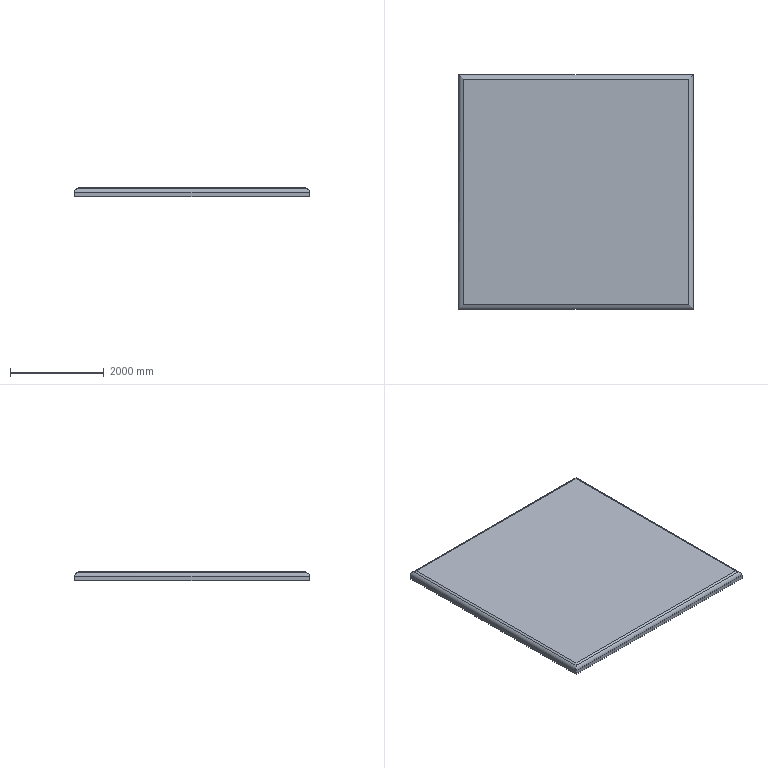Component | NX | 9_FLOOR | 1 solid | 14 faces | box 5000 x 5000 x 200 mm | volume 4937834897 mm3 | plane 10 | cylinder 4 | commonest cylinder face diameters 200 x4
STEP:
#1=CARTESIAN_POINT('',(0.,0.,0.));
#2=DIRECTION('',(0.,0.,1.));
#3=DIRECTION('',(1.,0.,0.));
#4=AXIS2_PLACEMENT_3D('',#1,#2,#3);
#5=CARTESIAN_POINT('',(3570.,2500.,-349.303));
#6=VERTEX_POINT('',#5);
#7=CARTESIAN_POINT('',(3570.,2500.,-437.5));
#8=VERTEX_POINT('',#7);
#9=CARTESIAN_POINT('',(3570.,2500.,-237.5));
#10=DIRECTION('',(0.,0.,-1.));
#11=VECTOR('',#10,1.);
#12=LINE('',#9,#11);
#13=CARTESIAN_POINT('',(3570.,-2500.,-237.5));
#14=DIRECTION('',(-1.,0.,0.));
#15=DIRECTION('',(-0.,-1.,0.));
#16=AXIS2_PLACEMENT_3D('',#13,#14,#15);
#17=PLANE('',#16);
#18=CARTESIAN_POINT('',(-5000.,0.));
#19=DIRECTION('',(0.,-1.));
#20=VECTOR('',#19,1.);
#21=LINE('',#18,#20);
#22=(GEOMETRIC_REPRESENTATION_CONTEXT(2)PARAMETRIC_REPRESENTATION_CONTEXT()REPRESENTATION_CONTEXT('',''));
#23=DEFINITIONAL_REPRESENTATION('',(#21),#22);
#24=PCURVE('',#17,#23);
#25=CARTESIAN_POINT('',(3570.,2500.,-237.5));
#26=DIRECTION('',(0.,-1.,0.));
#27=DIRECTION('',(0.,0.,1.));
#28=AXIS2_PLACEMENT_3D('',#25,#26,#27);
#29=PLANE('',#28);
#30=CARTESIAN_POINT('',(0.,0.));
#31=DIRECTION('',(-1.,0.));
#32=VECTOR('',#31,1.);
#33=LINE('',#30,#32);
#34=(GEOMETRIC_REPRESENTATION_CONTEXT(2)PARAMETRIC_REPRESENTATION_CONTEXT()REPRESENTATION_CONTEXT('',''));
#35=DEFINITIONAL_REPRESENTATION('',(#33),#34);
#36=PCURVE('',#29,#35);
#37=SURFACE_CURVE('',#12,(#24,#36),.PCURVE_S1.);
#38=EDGE_CURVE('',#6,#8,#37,.T.);
#39=ORIENTED_EDGE('',*,*,#38,.F.);
#40=CARTESIAN_POINT('',(3570.,-2500.,-349.303));
#41=VERTEX_POINT('',#40);
#42=CARTESIAN_POINT('',(3570.,-2500.,-349.303));
#43=DIRECTION('',(-0.,-1.,0.));
#44=VECTOR('',#43,1.);
#45=LINE('',#42,#44);
#46=CARTESIAN_POINT('',(0.,-111.803));
#47=DIRECTION('',(1.,0.));
#48=VECTOR('',#47,1.);
#49=LINE('',#46,#48);
#50=(GEOMETRIC_REPRESENTATION_CONTEXT(2)PARAMETRIC_REPRESENTATION_CONTEXT()REPRESENTATION_CONTEXT('',''));
#51=DEFINITIONAL_REPRESENTATION('',(#49),#50);
#52=PCURVE('',#17,#51);
#53=CARTESIAN_POINT('',(3470.,-2500.,-349.303));
#54=DIRECTION('',(0.,1.,0.));
#55=DIRECTION('',(-1.,0.,0.));
#56=AXIS2_PLACEMENT_3D('',#53,#54,#55);
#57=CYLINDRICAL_SURFACE('',#56,100.);
#58=CARTESIAN_POINT('',(3.142,0.));
#59=DIRECTION('',(0.,-1.));
#60=VECTOR('',#59,1.);
#61=LINE('',#58,#60);
#62=(GEOMETRIC_REPRESENTATION_CONTEXT(2)PARAMETRIC_REPRESENTATION_CONTEXT()REPRESENTATION_CONTEXT('',''));
#63=DEFINITIONAL_REPRESENTATION('',(#61),#62);
#64=PCURVE('',#57,#63);
#65=SURFACE_CURVE('',#45,(#52,#64),.PCURVE_S1.);
#66=EDGE_CURVE('',#6,#41,#65,.T.);
#67=ORIENTED_EDGE('',*,*,#66,.T.);
#68=CARTESIAN_POINT('',(3570.,-2500.,-437.5));
#69=VERTEX_POINT('',#68);
#70=CARTESIAN_POINT('',(3570.,-2500.,-237.5));
#71=DIRECTION('',(0.,0.,-1.));
#72=VECTOR('',#71,1.);
#73=LINE('',#70,#72);
#74=CARTESIAN_POINT('',(0.,0.));
#75=DIRECTION('',(0.,-1.));
#76=VECTOR('',#75,1.);
#77=LINE('',#74,#76);
#78=(GEOMETRIC_REPRESENTATION_CONTEXT(2)PARAMETRIC_REPRESENTATION_CONTEXT()REPRESENTATION_CONTEXT('',''));
#79=DEFINITIONAL_REPRESENTATION('',(#77),#78);
#80=PCURVE('',#17,#79);
#81=CARTESIAN_POINT('',(-1430.,-2500.,-237.5));
#82=DIRECTION('',(0.,1.,0.));
#83=DIRECTION('',(0.,0.,-1.));
#84=AXIS2_PLACEMENT_3D('',#81,#82,#83);
#85=PLANE('',#84);
#86=CARTESIAN_POINT('',(0.,-5000.));
#87=DIRECTION('',(1.,0.));
#88=VECTOR('',#87,1.);
#89=LINE('',#86,#88);
#90=(GEOMETRIC_REPRESENTATION_CONTEXT(2)PARAMETRIC_REPRESENTATION_CONTEXT()REPRESENTATION_CONTEXT('',''));
#91=DEFINITIONAL_REPRESENTATION('',(#89),#90);
#92=PCURVE('',#85,#91);
#93=SURFACE_CURVE('',#73,(#80,#92),.PCURVE_S1.);
#94=EDGE_CURVE('',#41,#69,#93,.T.);
#95=ORIENTED_EDGE('',*,*,#94,.T.);
#96=CARTESIAN_POINT('',(3570.,-2500.,-437.5));
#97=DIRECTION('',(0.,1.,0.));
#98=VECTOR('',#97,1.);
#99=LINE('',#96,#98);
#100=CARTESIAN_POINT('',(0.,-200.));
#101=DIRECTION('',(-1.,0.));
#102=VECTOR('',#101,1.);
#103=LINE('',#100,#102);
#104=(GEOMETRIC_REPRESENTATION_CONTEXT(2)PARAMETRIC_REPRESENTATION_CONTEXT()REPRESENTATION_CONTEXT('',''));
#105=DEFINITIONAL_REPRESENTATION('',(#103),#104);
#106=PCURVE('',#17,#105);
#107=CARTESIAN_POINT('',(1070.,-0.,-437.5));
#108=DIRECTION('',(0.,0.,1.));
#109=DIRECTION('',(-1.,0.,0.));
#110=AXIS2_PLACEMENT_3D('',#107,#108,#109);
#111=PLANE('',#110);
#112=CARTESIAN_POINT('',(-2500.,2500.));
#113=DIRECTION('',(-0.,-1.));
#114=VECTOR('',#113,1.);
#115=LINE('',#112,#114);
#116=(GEOMETRIC_REPRESENTATION_CONTEXT(2)PARAMETRIC_REPRESENTATION_CONTEXT()REPRESENTATION_CONTEXT('',''));
#117=DEFINITIONAL_REPRESENTATION('',(#115),#116);
#118=PCURVE('',#111,#117);
#119=SURFACE_CURVE('',#99,(#106,#118),.PCURVE_S1.);
#120=EDGE_CURVE('',#69,#8,#119,.T.);
#121=ORIENTED_EDGE('',*,*,#120,.T.);
#122=EDGE_LOOP('',(#39,#67,#95,#121));
#123=FACE_BOUND('',#122,.T.);
#124=ADVANCED_FACE('',(#123),#17,.F.);
#125=CARTESIAN_POINT('',(-1430.,2500.,-349.303));
#126=VERTEX_POINT('',#125);
#127=CARTESIAN_POINT('',(-1430.,2500.,-437.5));
#128=VERTEX_POINT('',#127);
#129=CARTESIAN_POINT('',(-1430.,2500.,-237.5));
#130=DIRECTION('',(0.,0.,-1.));
#131=VECTOR('',#130,1.);
#132=LINE('',#129,#131);
#133=CARTESIAN_POINT('',(0.,5000.));
#134=DIRECTION('',(-1.,0.));
#135=VECTOR('',#134,1.);
#136=LINE('',#133,#135);
#137=(GEOMETRIC_REPRESENTATION_CONTEXT(2)PARAMETRIC_REPRESENTATION_CONTEXT()REPRESENTATION_CONTEXT('',''));
#138=DEFINITIONAL_REPRESENTATION('',(#136),#137);
#139=PCURVE('',#29,#138);
#140=CARTESIAN_POINT('',(-1430.,2500.,-237.5));
#141=DIRECTION('',(1.,-0.,0.));
#142=DIRECTION('',(0.,1.,0.));
#143=AXIS2_PLACEMENT_3D('',#140,#141,#142);
#144=PLANE('',#143);
#145=CARTESIAN_POINT('',(0.,0.));
#146=DIRECTION('',(0.,-1.));
#147=VECTOR('',#146,1.);
#148=LINE('',#145,#147);
#149=(GEOMETRIC_REPRESENTATION_CONTEXT(2)PARAMETRIC_REPRESENTATION_CONTEXT()REPRESENTATION_CONTEXT('',''));
#150=DEFINITIONAL_REPRESENTATION('',(#148),#149);
#151=PCURVE('',#144,#150);
#152=SURFACE_CURVE('',#132,(#139,#151),.PCURVE_S1.);
#153=EDGE_CURVE('',#126,#128,#152,.T.);
#154=ORIENTED_EDGE('',*,*,#153,.F.);
#155=CARTESIAN_POINT('',(3570.,2500.,-349.303));
#156=DIRECTION('',(1.,0.,0.));
#157=VECTOR('',#156,1.);
#158=LINE('',#155,#157);
#159=CARTESIAN_POINT('',(-111.803,0.));
#160=DIRECTION('',(0.,-1.));
#161=VECTOR('',#160,1.);
#162=LINE('',#159,#161);
#163=(GEOMETRIC_REPRESENTATION_CONTEXT(2)PARAMETRIC_REPRESENTATION_CONTEXT()REPRESENTATION_CONTEXT('',''));
#164=DEFINITIONAL_REPRESENTATION('',(#162),#163);
#165=PCURVE('',#29,#164);
#166=CARTESIAN_POINT('',(3570.,2400.,-349.303));
#167=DIRECTION('',(-1.,0.,0.));
#168=DIRECTION('',(0.,0.,-1.));
#169=AXIS2_PLACEMENT_3D('',#166,#167,#168);
#170=CYLINDRICAL_SURFACE('',#169,100.);
#171=CARTESIAN_POINT('',(4.712,0.));
#172=DIRECTION('',(0.,-1.));
#173=VECTOR('',#172,1.);
#174=LINE('',#171,#173);
#175=(GEOMETRIC_REPRESENTATION_CONTEXT(2)PARAMETRIC_REPRESENTATION_CONTEXT()REPRESENTATION_CONTEXT('',''));
#176=DEFINITIONAL_REPRESENTATION('',(#174),#175);
#177=PCURVE('',#170,#176);
#178=SURFACE_CURVE('',#158,(#165,#177),.PCURVE_S1.);
#179=EDGE_CURVE('',#126,#6,#178,.T.);
#180=ORIENTED_EDGE('',*,*,#179,.T.);
#181=ORIENTED_EDGE('',*,*,#38,.T.);
#182=CARTESIAN_POINT('',(3570.,2500.,-437.5));
#183=DIRECTION('',(-1.,0.,0.));
#184=VECTOR('',#183,1.);
#185=LINE('',#182,#184);
#186=CARTESIAN_POINT('',(-200.,0.));
#187=DIRECTION('',(0.,1.));
#188=VECTOR('',#187,1.);
#189=LINE('',#186,#188);
#190=(GEOMETRIC_REPRESENTATION_CONTEXT(2)PARAMETRIC_REPRESENTATION_CONTEXT()REPRESENTATION_CONTEXT('',''));
#191=DEFINITIONAL_REPRESENTATION('',(#189),#190);
#192=PCURVE('',#29,#191);
#193=CARTESIAN_POINT('',(-2500.,-2500.));
#194=DIRECTION('',(1.,0.));
#195=VECTOR('',#194,1.);
#196=LINE('',#193,#195);
#197=(GEOMETRIC_REPRESENTATION_CONTEXT(2)PARAMETRIC_REPRESENTATION_CONTEXT()REPRESENTATION_CONTEXT('',''));
#198=DEFINITIONAL_REPRESENTATION('',(#196),#197);
#199=PCURVE('',#111,#198);
#200=SURFACE_CURVE('',#185,(#192,#199),.PCURVE_S1.);
#201=EDGE_CURVE('',#8,#128,#200,.T.);
#202=ORIENTED_EDGE('',*,*,#201,.T.);
#203=EDGE_LOOP('',(#154,#180,#181,#202));
#204=FACE_BOUND('',#203,.T.);
#205=ADVANCED_FACE('',(#204),#29,.F.);
#206=CARTESIAN_POINT('',(-1430.,-2500.,-349.303));
#207=VERTEX_POINT('',#206);
#208=CARTESIAN_POINT('',(-1430.,-2500.,-437.5));
#209=VERTEX_POINT('',#208);
#210=CARTESIAN_POINT('',(-1430.,-2500.,-237.5));
#211=DIRECTION('',(0.,0.,-1.));
#212=VECTOR('',#211,1.);
#213=LINE('',#210,#212);
#214=CARTESIAN_POINT('',(-5000.,0.));
#215=DIRECTION('',(0.,-1.));
#216=VECTOR('',#215,1.);
#217=LINE('',#214,#216);
#218=(GEOMETRIC_REPRESENTATION_CONTEXT(2)PARAMETRIC_REPRESENTATION_CONTEXT()REPRESENTATION_CONTEXT('',''));
#219=DEFINITIONAL_REPRESENTATION('',(#217),#218);
#220=PCURVE('',#144,#219);
#221=CARTESIAN_POINT('',(0.,0.));
#222=DIRECTION('',(1.,0.));
#223=VECTOR('',#222,1.);
#224=LINE('',#221,#223);
#225=(GEOMETRIC_REPRESENTATION_CONTEXT(2)PARAMETRIC_REPRESENTATION_CONTEXT()REPRESENTATION_CONTEXT('',''));
#226=DEFINITIONAL_REPRESENTATION('',(#224),#225);
#227=PCURVE('',#85,#226);
#228=SURFACE_CURVE('',#213,(#220,#227),.PCURVE_S1.);
#229=EDGE_CURVE('',#207,#209,#228,.T.);
#230=ORIENTED_EDGE('',*,*,#229,.F.);
#231=CARTESIAN_POINT('',(-1430.,2500.,-349.303));
#232=DIRECTION('',(0.,1.,0.));
#233=VECTOR('',#232,1.);
#234=LINE('',#231,#233);
#235=CARTESIAN_POINT('',(0.,-111.803));
#236=DIRECTION('',(1.,0.));
#237=VECTOR('',#236,1.);
#238=LINE('',#235,#237);
#239=(GEOMETRIC_REPRESENTATION_CONTEXT(2)PARAMETRIC_REPRESENTATION_CONTEXT()REPRESENTATION_CONTEXT('',''));
#240=DEFINITIONAL_REPRESENTATION('',(#238),#239);
#241=PCURVE('',#144,#240);
#242=CARTESIAN_POINT('',(-1330.,2500.,-349.303));
#243=DIRECTION('',(-0.,-1.,0.));
#244=DIRECTION('',(1.,-0.,0.));
#245=AXIS2_PLACEMENT_3D('',#242,#243,#244);
#246=CYLINDRICAL_SURFACE('',#245,100.);
#247=CARTESIAN_POINT('',(3.142,0.));
#248=DIRECTION('',(0.,-1.));
#249=VECTOR('',#248,1.);
#250=LINE('',#247,#249);
#251=(GEOMETRIC_REPRESENTATION_CONTEXT(2)PARAMETRIC_REPRESENTATION_CONTEXT()REPRESENTATION_CONTEXT('',''));
#252=DEFINITIONAL_REPRESENTATION('',(#250),#251);
#253=PCURVE('',#246,#252);
#254=SURFACE_CURVE('',#234,(#241,#253),.PCURVE_S1.);
#255=EDGE_CURVE('',#207,#126,#254,.T.);
#256=ORIENTED_EDGE('',*,*,#255,.T.);
#257=ORIENTED_EDGE('',*,*,#153,.T.);
#258=CARTESIAN_POINT('',(-1430.,2500.,-437.5));
#259=DIRECTION('',(-0.,-1.,0.));
#260=VECTOR('',#259,1.);
#261=LINE('',#258,#260);
#262=CARTESIAN_POINT('',(0.,-200.));
#263=DIRECTION('',(-1.,0.));
#264=VECTOR('',#263,1.);
#265=LINE('',#262,#264);
#266=(GEOMETRIC_REPRESENTATION_CONTEXT(2)PARAMETRIC_REPRESENTATION_CONTEXT()REPRESENTATION_CONTEXT('',''));
#267=DEFINITIONAL_REPRESENTATION('',(#265),#266);
#268=PCURVE('',#144,#267);
#269=CARTESIAN_POINT('',(2500.,-2500.));
#270=DIRECTION('',(0.,1.));
#271=VECTOR('',#270,1.);
#272=LINE('',#269,#271);
#273=(GEOMETRIC_REPRESENTATION_CONTEXT(2)PARAMETRIC_REPRESENTATION_CONTEXT()REPRESENTATION_CONTEXT('',''));
#274=DEFINITIONAL_REPRESENTATION('',(#272),#273);
#275=PCURVE('',#111,#274);
#276=SURFACE_CURVE('',#261,(#268,#275),.PCURVE_S1.);
#277=EDGE_CURVE('',#128,#209,#276,.T.);
#278=ORIENTED_EDGE('',*,*,#277,.T.);
#279=EDGE_LOOP('',(#230,#256,#257,#278));
#280=FACE_BOUND('',#279,.T.);
#281=ADVANCED_FACE('',(#280),#144,.F.);
#282=ORIENTED_EDGE('',*,*,#94,.F.);
#283=CARTESIAN_POINT('',(-1430.,-2500.,-349.303));
#284=DIRECTION('',(-1.,0.,0.));
#285=VECTOR('',#284,1.);
#286=LINE('',#283,#285);
#287=CARTESIAN_POINT('',(111.803,0.));
#288=DIRECTION('',(0.,1.));
#289=VECTOR('',#288,1.);
#290=LINE('',#287,#289);
#291=(GEOMETRIC_REPRESENTATION_CONTEXT(2)PARAMETRIC_REPRESENTATION_CONTEXT()REPRESENTATION_CONTEXT('',''));
#292=DEFINITIONAL_REPRESENTATION('',(#290),#291);
#293=PCURVE('',#85,#292);
#294=CARTESIAN_POINT('',(-1430.,-2400.,-349.303));
#295=DIRECTION('',(1.,0.,0.));
#296=DIRECTION('',(0.,0.,1.));
#297=AXIS2_PLACEMENT_3D('',#294,#295,#296);
#298=CYLINDRICAL_SURFACE('',#297,100.);
#299=CARTESIAN_POINT('',(1.571,0.));
#300=DIRECTION('',(0.,-1.));
#301=VECTOR('',#300,1.);
#302=LINE('',#299,#301);
#303=(GEOMETRIC_REPRESENTATION_CONTEXT(2)PARAMETRIC_REPRESENTATION_CONTEXT()REPRESENTATION_CONTEXT('',''));
#304=DEFINITIONAL_REPRESENTATION('',(#302),#303);
#305=PCURVE('',#298,#304);
#306=SURFACE_CURVE('',#286,(#293,#305),.PCURVE_S1.);
#307=EDGE_CURVE('',#41,#207,#306,.T.);
#308=ORIENTED_EDGE('',*,*,#307,.T.);
#309=ORIENTED_EDGE('',*,*,#229,.T.);
#310=CARTESIAN_POINT('',(-1430.,-2500.,-437.5));
#311=DIRECTION('',(1.,0.,0.));
#312=VECTOR('',#311,1.);
#313=LINE('',#310,#312);
#314=CARTESIAN_POINT('',(200.,0.));
#315=DIRECTION('',(0.,-1.));
#316=VECTOR('',#315,1.);
#317=LINE('',#314,#316);
#318=(GEOMETRIC_REPRESENTATION_CONTEXT(2)PARAMETRIC_REPRESENTATION_CONTEXT()REPRESENTATION_CONTEXT('',''));
#319=DEFINITIONAL_REPRESENTATION('',(#317),#318);
#320=PCURVE('',#85,#319);
#321=CARTESIAN_POINT('',(2500.,2500.));
#322=DIRECTION('',(-1.,0.));
#323=VECTOR('',#322,1.);
#324=LINE('',#321,#323);
#325=(GEOMETRIC_REPRESENTATION_CONTEXT(2)PARAMETRIC_REPRESENTATION_CONTEXT()REPRESENTATION_CONTEXT('',''));
#326=DEFINITIONAL_REPRESENTATION('',(#324),#325);
#327=PCURVE('',#111,#326);
#328=SURFACE_CURVE('',#313,(#320,#327),.PCURVE_S1.);
#329=EDGE_CURVE('',#209,#69,#328,.T.);
#330=ORIENTED_EDGE('',*,*,#329,.T.);
#331=EDGE_LOOP('',(#282,#308,#309,#330));
#332=FACE_BOUND('',#331,.T.);
#333=ADVANCED_FACE('',(#332),#85,.F.);
#334=CARTESIAN_POINT('',(3470.,2400.,-237.5));
#335=VERTEX_POINT('',#334);
#336=CARTESIAN_POINT('',(-1330.,2400.,-237.5));
#337=VERTEX_POINT('',#336);
#338=CARTESIAN_POINT('',(-1430.,2400.,-237.5));
#339=DIRECTION('',(-1.,0.,0.));
#340=VECTOR('',#339,1.);
#341=LINE('',#338,#340);
#342=CARTESIAN_POINT('',(1070.,-0.,-237.5));
#343=DIRECTION('',(0.,0.,1.));
#344=DIRECTION('',(-1.,0.,0.));
#345=AXIS2_PLACEMENT_3D('',#342,#343,#344);
#346=PLANE('',#345);
#347=CARTESIAN_POINT('',(2500.,-2400.));
#348=DIRECTION('',(1.,0.));
#349=VECTOR('',#348,1.);
#350=LINE('',#347,#349);
#351=(GEOMETRIC_REPRESENTATION_CONTEXT(2)PARAMETRIC_REPRESENTATION_CONTEXT()REPRESENTATION_CONTEXT('',''));
#352=DEFINITIONAL_REPRESENTATION('',(#350),#351);
#353=PCURVE('',#346,#352);
#354=CARTESIAN_POINT('',(1070.,2400.,-237.5));
#355=DIRECTION('',(0.,0.4472,0.8944));
#356=DIRECTION('',(1.,0.,0.));
#357=AXIS2_PLACEMENT_3D('',#354,#355,#356);
#358=PLANE('',#357);
#359=CARTESIAN_POINT('',(-2500.,0.));
#360=DIRECTION('',(-1.,0.));
#361=VECTOR('',#360,1.);
#362=LINE('',#359,#361);
#363=(GEOMETRIC_REPRESENTATION_CONTEXT(2)PARAMETRIC_REPRESENTATION_CONTEXT()REPRESENTATION_CONTEXT('',''));
#364=DEFINITIONAL_REPRESENTATION('',(#362),#363);
#365=PCURVE('',#358,#364);
#366=SURFACE_CURVE('',#341,(#353,#365),.PCURVE_S1.);
#367=EDGE_CURVE('',#335,#337,#366,.T.);
#368=ORIENTED_EDGE('',*,*,#367,.T.);
#369=CARTESIAN_POINT('',(-1330.,-2400.,-237.5));
#370=VERTEX_POINT('',#369);
#371=CARTESIAN_POINT('',(-1330.,-2500.,-237.5));
#372=DIRECTION('',(-0.,-1.,0.));
#373=VECTOR('',#372,1.);
#374=LINE('',#371,#373);
#375=CARTESIAN_POINT('',(2400.,2500.));
#376=DIRECTION('',(0.,1.));
#377=VECTOR('',#376,1.);
#378=LINE('',#375,#377);
#379=(GEOMETRIC_REPRESENTATION_CONTEXT(2)PARAMETRIC_REPRESENTATION_CONTEXT()REPRESENTATION_CONTEXT('',''));
#380=DEFINITIONAL_REPRESENTATION('',(#378),#379);
#381=PCURVE('',#346,#380);
#382=CARTESIAN_POINT('',(-1330.,0.,-237.5));
#383=DIRECTION('',(-0.4472,0.,0.8944));
#384=DIRECTION('',(0.,1.,-0.));
#385=AXIS2_PLACEMENT_3D('',#382,#383,#384);
#386=PLANE('',#385);
#387=CARTESIAN_POINT('',(-2500.,-0.));
#388=DIRECTION('',(-1.,0.));
#389=VECTOR('',#388,1.);
#390=LINE('',#387,#389);
#391=(GEOMETRIC_REPRESENTATION_CONTEXT(2)PARAMETRIC_REPRESENTATION_CONTEXT()REPRESENTATION_CONTEXT('',''));
#392=DEFINITIONAL_REPRESENTATION('',(#390),#391);
#393=PCURVE('',#386,#392);
#394=SURFACE_CURVE('',#374,(#381,#393),.PCURVE_S1.);
#395=EDGE_CURVE('',#337,#370,#394,.T.);
#396=ORIENTED_EDGE('',*,*,#395,.T.);
#397=CARTESIAN_POINT('',(3470.,-2400.,-237.5));
#398=VERTEX_POINT('',#397);
#399=CARTESIAN_POINT('',(3570.,-2400.,-237.5));
#400=DIRECTION('',(1.,0.,0.));
#401=VECTOR('',#400,1.);
#402=LINE('',#399,#401);
#403=CARTESIAN_POINT('',(-2500.,2400.));
#404=DIRECTION('',(-1.,0.));
#405=VECTOR('',#404,1.);
#406=LINE('',#403,#405);
#407=(GEOMETRIC_REPRESENTATION_CONTEXT(2)PARAMETRIC_REPRESENTATION_CONTEXT()REPRESENTATION_CONTEXT('',''));
#408=DEFINITIONAL_REPRESENTATION('',(#406),#407);
#409=PCURVE('',#346,#408);
#410=CARTESIAN_POINT('',(1070.,-2400.,-237.5));
#411=DIRECTION('',(0.,-0.4472,0.8944));
#412=DIRECTION('',(-1.,0.,0.));
#413=AXIS2_PLACEMENT_3D('',#410,#411,#412);
#414=PLANE('',#413);
#415=CARTESIAN_POINT('',(-2500.,0.));
#416=DIRECTION('',(-1.,0.));
#417=VECTOR('',#416,1.);
#418=LINE('',#415,#417);
#419=(GEOMETRIC_REPRESENTATION_CONTEXT(2)PARAMETRIC_REPRESENTATION_CONTEXT()REPRESENTATION_CONTEXT('',''));
#420=DEFINITIONAL_REPRESENTATION('',(#418),#419);
#421=PCURVE('',#414,#420);
#422=SURFACE_CURVE('',#402,(#409,#421),.PCURVE_S1.);
#423=EDGE_CURVE('',#370,#398,#422,.T.);
#424=ORIENTED_EDGE('',*,*,#423,.T.);
#425=CARTESIAN_POINT('',(3470.,2500.,-237.5));
#426=DIRECTION('',(0.,1.,0.));
#427=VECTOR('',#426,1.);
#428=LINE('',#425,#427);
#429=CARTESIAN_POINT('',(-2400.,-2500.));
#430=DIRECTION('',(-0.,-1.));
#431=VECTOR('',#430,1.);
#432=LINE('',#429,#431);
#433=(GEOMETRIC_REPRESENTATION_CONTEXT(2)PARAMETRIC_REPRESENTATION_CONTEXT()REPRESENTATION_CONTEXT('',''));
#434=DEFINITIONAL_REPRESENTATION('',(#432),#433);
#435=PCURVE('',#346,#434);
#436=CARTESIAN_POINT('',(3470.,-0.,-237.5));
#437=DIRECTION('',(0.4472,-0.,0.8944));
#438=DIRECTION('',(-0.,-1.,0.));
#439=AXIS2_PLACEMENT_3D('',#436,#437,#438);
#440=PLANE('',#439);
#441=CARTESIAN_POINT('',(-2500.,-0.));
#442=DIRECTION('',(-1.,-0.));
#443=VECTOR('',#442,1.);
#444=LINE('',#441,#443);
#445=(GEOMETRIC_REPRESENTATION_CONTEXT(2)PARAMETRIC_REPRESENTATION_CONTEXT()REPRESENTATION_CONTEXT('',''));
#446=DEFINITIONAL_REPRESENTATION('',(#444),#445);
#447=PCURVE('',#440,#446);
#448=SURFACE_CURVE('',#428,(#435,#447),.PCURVE_S1.);
#449=EDGE_CURVE('',#398,#335,#448,.T.);
#450=ORIENTED_EDGE('',*,*,#449,.T.);
#451=EDGE_LOOP('',(#368,#396,#424,#450));
#452=FACE_BOUND('',#451,.T.);
#453=ADVANCED_FACE('',(#452),#346,.T.);
#454=ORIENTED_EDGE('',*,*,#120,.F.);
#455=ORIENTED_EDGE('',*,*,#329,.F.);
#456=ORIENTED_EDGE('',*,*,#277,.F.);
#457=ORIENTED_EDGE('',*,*,#201,.F.);
#458=EDGE_LOOP('',(#454,#455,#456,#457));
#459=FACE_BOUND('',#458,.T.);
#460=ADVANCED_FACE('',(#459),#111,.F.);
#461=CARTESIAN_POINT('',(3514.721,-2444.721,-259.861));
#462=VERTEX_POINT('',#461);
#463=CARTESIAN_POINT('',(2403.333,-1333.333,295.833));
#464=DIRECTION('',(-0.6667,0.6667,0.3333));
#465=VECTOR('',#464,1.);
#466=LINE('',#463,#465);
#467=CARTESIAN_POINT('',(1333.333,-1192.57));
#468=DIRECTION('',(-0.6667,-0.7454));
#469=VECTOR('',#468,1.);
#470=LINE('',#467,#469);
#471=(GEOMETRIC_REPRESENTATION_CONTEXT(2)PARAMETRIC_REPRESENTATION_CONTEXT()REPRESENTATION_CONTEXT('',''));
#472=DEFINITIONAL_REPRESENTATION('',(#470),#471);
#473=PCURVE('',#440,#472);
#474=CARTESIAN_POINT('',(-1333.333,-1192.57));
#475=DIRECTION('',(0.6667,-0.7454));
#476=VECTOR('',#475,1.);
#477=LINE('',#474,#476);
#478=(GEOMETRIC_REPRESENTATION_CONTEXT(2)PARAMETRIC_REPRESENTATION_CONTEXT()REPRESENTATION_CONTEXT('',''));
#479=DEFINITIONAL_REPRESENTATION('',(#477),#478);
#480=PCURVE('',#414,#479);
#481=SURFACE_CURVE('',#466,(#473,#480),.PCURVE_S1.);
#482=EDGE_CURVE('',#462,#398,#481,.T.);
#483=ORIENTED_EDGE('',*,*,#482,.F.);
#484=CARTESIAN_POINT('',(3514.721,2444.721,-259.861));
#485=VERTEX_POINT('',#484);
#486=CARTESIAN_POINT('',(3514.721,2500.,-259.861));
#487=DIRECTION('',(0.,1.,0.));
#488=VECTOR('',#487,1.);
#489=LINE('',#486,#488);
#490=CARTESIAN_POINT('',(-2500.,50.));
#491=DIRECTION('',(-1.,-0.));
#492=VECTOR('',#491,1.);
#493=LINE('',#490,#492);
#494=(GEOMETRIC_REPRESENTATION_CONTEXT(2)PARAMETRIC_REPRESENTATION_CONTEXT()REPRESENTATION_CONTEXT('',''));
#495=DEFINITIONAL_REPRESENTATION('',(#493),#494);
#496=PCURVE('',#440,#495);
#497=CARTESIAN_POINT('',(2.034,5000.));
#498=DIRECTION('',(0.,1.));
#499=VECTOR('',#498,1.);
#500=LINE('',#497,#499);
#501=(GEOMETRIC_REPRESENTATION_CONTEXT(2)PARAMETRIC_REPRESENTATION_CONTEXT()REPRESENTATION_CONTEXT('',''));
#502=DEFINITIONAL_REPRESENTATION('',(#500),#501);
#503=PCURVE('',#57,#502);
#504=SURFACE_CURVE('',#489,(#496,#503),.PCURVE_S1.);
#505=EDGE_CURVE('',#462,#485,#504,.T.);
#506=ORIENTED_EDGE('',*,*,#505,.T.);
#507=CARTESIAN_POINT('',(2403.333,1333.333,295.833));
#508=DIRECTION('',(0.6667,0.6667,-0.3333));
#509=VECTOR('',#508,1.);
#510=LINE('',#507,#509);
#511=CARTESIAN_POINT('',(-1333.333,-1192.57));
#512=DIRECTION('',(-0.6667,0.7454));
#513=VECTOR('',#512,1.);
#514=LINE('',#511,#513);
#515=(GEOMETRIC_REPRESENTATION_CONTEXT(2)PARAMETRIC_REPRESENTATION_CONTEXT()REPRESENTATION_CONTEXT('',''));
#516=DEFINITIONAL_REPRESENTATION('',(#514),#515);
#517=PCURVE('',#440,#516);
#518=CARTESIAN_POINT('',(1333.333,-1192.57));
#519=DIRECTION('',(0.6667,0.7454));
#520=VECTOR('',#519,1.);
#521=LINE('',#518,#520);
#522=(GEOMETRIC_REPRESENTATION_CONTEXT(2)PARAMETRIC_REPRESENTATION_CONTEXT()REPRESENTATION_CONTEXT('',''));
#523=DEFINITIONAL_REPRESENTATION('',(#521),#522);
#524=PCURVE('',#358,#523);
#525=SURFACE_CURVE('',#510,(#517,#524),.PCURVE_S1.);
#526=EDGE_CURVE('',#335,#485,#525,.T.);
#527=ORIENTED_EDGE('',*,*,#526,.F.);
#528=ORIENTED_EDGE('',*,*,#449,.F.);
#529=EDGE_LOOP('',(#483,#506,#527,#528));
#530=FACE_BOUND('',#529,.T.);
#531=ADVANCED_FACE('',(#530),#440,.T.);
#532=ORIENTED_EDGE('',*,*,#526,.T.);
#533=CARTESIAN_POINT('',(-1374.721,2444.721,-259.861));
#534=VERTEX_POINT('',#533);
#535=CARTESIAN_POINT('',(-1430.,2444.721,-259.861));
#536=DIRECTION('',(-1.,0.,0.));
#537=VECTOR('',#536,1.);
#538=LINE('',#535,#537);
#539=CARTESIAN_POINT('',(-2500.,50.));
#540=DIRECTION('',(-1.,0.));
#541=VECTOR('',#540,1.);
#542=LINE('',#539,#541);
#543=(GEOMETRIC_REPRESENTATION_CONTEXT(2)PARAMETRIC_REPRESENTATION_CONTEXT()REPRESENTATION_CONTEXT('',''));
#544=DEFINITIONAL_REPRESENTATION('',(#542),#543);
#545=PCURVE('',#358,#544);
#546=CARTESIAN_POINT('',(3.605,5000.));
#547=DIRECTION('',(0.,1.));
#548=VECTOR('',#547,1.);
#549=LINE('',#546,#548);
#550=(GEOMETRIC_REPRESENTATION_CONTEXT(2)PARAMETRIC_REPRESENTATION_CONTEXT()REPRESENTATION_CONTEXT('',''));
#551=DEFINITIONAL_REPRESENTATION('',(#549),#550);
#552=PCURVE('',#170,#551);
#553=SURFACE_CURVE('',#538,(#545,#552),.PCURVE_S1.);
#554=EDGE_CURVE('',#485,#534,#553,.T.);
#555=ORIENTED_EDGE('',*,*,#554,.T.);
#556=CARTESIAN_POINT('',(-263.333,1333.333,295.833));
#557=DIRECTION('',(-0.6667,0.6667,-0.3333));
#558=VECTOR('',#557,1.);
#559=LINE('',#556,#558);
#560=CARTESIAN_POINT('',(-1333.333,-1192.57));
#561=DIRECTION('',(-0.6667,0.7454));
#562=VECTOR('',#561,1.);
#563=LINE('',#560,#562);
#564=(GEOMETRIC_REPRESENTATION_CONTEXT(2)PARAMETRIC_REPRESENTATION_CONTEXT()REPRESENTATION_CONTEXT('',''));
#565=DEFINITIONAL_REPRESENTATION('',(#563),#564);
#566=PCURVE('',#358,#565);
#567=CARTESIAN_POINT('',(1333.333,-1192.57));
#568=DIRECTION('',(0.6667,0.7454));
#569=VECTOR('',#568,1.);
#570=LINE('',#567,#569);
#571=(GEOMETRIC_REPRESENTATION_CONTEXT(2)PARAMETRIC_REPRESENTATION_CONTEXT()REPRESENTATION_CONTEXT('',''));
#572=DEFINITIONAL_REPRESENTATION('',(#570),#571);
#573=PCURVE('',#386,#572);
#574=SURFACE_CURVE('',#559,(#566,#573),.PCURVE_S1.);
#575=EDGE_CURVE('',#337,#534,#574,.T.);
#576=ORIENTED_EDGE('',*,*,#575,.F.);
#577=ORIENTED_EDGE('',*,*,#367,.F.);
#578=EDGE_LOOP('',(#532,#555,#576,#577));
#579=FACE_BOUND('',#578,.T.);
#580=ADVANCED_FACE('',(#579),#358,.T.);
#581=CARTESIAN_POINT('',(-1374.721,-2444.721,-259.861));
#582=VERTEX_POINT('',#581);
#583=CARTESIAN_POINT('',(-263.333,-1333.333,295.833));
#584=DIRECTION('',(0.6667,0.6667,0.3333));
#585=VECTOR('',#584,1.);
#586=LINE('',#583,#585);
#587=CARTESIAN_POINT('',(1333.333,-1192.57));
#588=DIRECTION('',(-0.6667,-0.7454));
#589=VECTOR('',#588,1.);
#590=LINE('',#587,#589);
#591=(GEOMETRIC_REPRESENTATION_CONTEXT(2)PARAMETRIC_REPRESENTATION_CONTEXT()REPRESENTATION_CONTEXT('',''));
#592=DEFINITIONAL_REPRESENTATION('',(#590),#591);
#593=PCURVE('',#414,#592);
#594=CARTESIAN_POINT('',(-1333.333,-1192.57));
#595=DIRECTION('',(0.6667,-0.7454));
#596=VECTOR('',#595,1.);
#597=LINE('',#594,#596);
#598=(GEOMETRIC_REPRESENTATION_CONTEXT(2)PARAMETRIC_REPRESENTATION_CONTEXT()REPRESENTATION_CONTEXT('',''));
#599=DEFINITIONAL_REPRESENTATION('',(#597),#598);
#600=PCURVE('',#386,#599);
#601=SURFACE_CURVE('',#586,(#593,#600),.PCURVE_S1.);
#602=EDGE_CURVE('',#582,#370,#601,.T.);
#603=ORIENTED_EDGE('',*,*,#602,.F.);
#604=CARTESIAN_POINT('',(3570.,-2444.721,-259.861));
#605=DIRECTION('',(1.,0.,0.));
#606=VECTOR('',#605,1.);
#607=LINE('',#604,#606);
#608=CARTESIAN_POINT('',(-2500.,50.));
#609=DIRECTION('',(-1.,0.));
#610=VECTOR('',#609,1.);
#611=LINE('',#608,#610);
#612=(GEOMETRIC_REPRESENTATION_CONTEXT(2)PARAMETRIC_REPRESENTATION_CONTEXT()REPRESENTATION_CONTEXT('',''));
#613=DEFINITIONAL_REPRESENTATION('',(#611),#612);
#614=PCURVE('',#414,#613);
#615=CARTESIAN_POINT('',(0.4636,5000.));
#616=DIRECTION('',(0.,1.));
#617=VECTOR('',#616,1.);
#618=LINE('',#615,#617);
#619=(GEOMETRIC_REPRESENTATION_CONTEXT(2)PARAMETRIC_REPRESENTATION_CONTEXT()REPRESENTATION_CONTEXT('',''));
#620=DEFINITIONAL_REPRESENTATION('',(#618),#619);
#621=PCURVE('',#298,#620);
#622=SURFACE_CURVE('',#607,(#614,#621),.PCURVE_S1.);
#623=EDGE_CURVE('',#582,#462,#622,.T.);
#624=ORIENTED_EDGE('',*,*,#623,.T.);
#625=ORIENTED_EDGE('',*,*,#482,.T.);
#626=ORIENTED_EDGE('',*,*,#423,.F.);
#627=EDGE_LOOP('',(#603,#624,#625,#626));
#628=FACE_BOUND('',#627,.T.);
#629=ADVANCED_FACE('',(#628),#414,.T.);
#630=ORIENTED_EDGE('',*,*,#575,.T.);
#631=CARTESIAN_POINT('',(-1374.721,-2500.,-259.861));
#632=DIRECTION('',(-0.,-1.,0.));
#633=VECTOR('',#632,1.);
#634=LINE('',#631,#633);
#635=CARTESIAN_POINT('',(-2500.,50.));
#636=DIRECTION('',(-1.,0.));
#637=VECTOR('',#636,1.);
#638=LINE('',#635,#637);
#639=(GEOMETRIC_REPRESENTATION_CONTEXT(2)PARAMETRIC_REPRESENTATION_CONTEXT()REPRESENTATION_CONTEXT('',''));
#640=DEFINITIONAL_REPRESENTATION('',(#638),#639);
#641=PCURVE('',#386,#640);
#642=CARTESIAN_POINT('',(2.034,5000.));
#643=DIRECTION('',(0.,1.));
#644=VECTOR('',#643,1.);
#645=LINE('',#642,#644);
#646=(GEOMETRIC_REPRESENTATION_CONTEXT(2)PARAMETRIC_REPRESENTATION_CONTEXT()REPRESENTATION_CONTEXT('',''));
#647=DEFINITIONAL_REPRESENTATION('',(#645),#646);
#648=PCURVE('',#246,#647);
#649=SURFACE_CURVE('',#634,(#641,#648),.PCURVE_S1.);
#650=EDGE_CURVE('',#534,#582,#649,.T.);
#651=ORIENTED_EDGE('',*,*,#650,.T.);
#652=ORIENTED_EDGE('',*,*,#602,.T.);
#653=ORIENTED_EDGE('',*,*,#395,.F.);
#654=EDGE_LOOP('',(#630,#651,#652,#653));
#655=FACE_BOUND('',#654,.T.);
#656=ADVANCED_FACE('',(#655),#386,.T.);
#657=CARTESIAN_POINT('',(-1330.,-2400.,-349.303));
#658=DIRECTION('',(0.7071,-0.7071,0.));
#659=DIRECTION('',(-0.7071,-0.7071,0.));
#660=AXIS2_PLACEMENT_3D('',#657,#658,#659);
#661=ELLIPSE('',#660,141.421,100.);
#662=CARTESIAN_POINT('',(2.034,4944.721));
#663=CARTESIAN_POINT('',(2.051,4946.222));
#664=CARTESIAN_POINT('',(2.085,4949.185));
#665=CARTESIAN_POINT('',(2.135,4953.505));
#666=CARTESIAN_POINT('',(2.185,4957.689));
#667=CARTESIAN_POINT('',(2.236,4961.728));
#668=CARTESIAN_POINT('',(2.286,4965.61));
#669=CARTESIAN_POINT('',(2.336,4969.326));
#670=CARTESIAN_POINT('',(2.387,4972.867));
#671=CARTESIAN_POINT('',(2.437,4976.223));
#672=CARTESIAN_POINT('',(2.487,4979.386));
#673=CARTESIAN_POINT('',(2.538,4982.348));
#674=CARTESIAN_POINT('',(2.588,4985.101));
#675=CARTESIAN_POINT('',(2.638,4987.639));
#676=CARTESIAN_POINT('',(2.689,4989.955));
#677=CARTESIAN_POINT('',(2.739,4992.043));
#678=CARTESIAN_POINT('',(2.789,4993.899));
#679=CARTESIAN_POINT('',(2.84,4995.516));
#680=CARTESIAN_POINT('',(2.89,4996.892));
#681=CARTESIAN_POINT('',(2.94,4998.022));
#682=CARTESIAN_POINT('',(2.991,4998.904));
#683=CARTESIAN_POINT('',(3.041,4999.536));
#684=CARTESIAN_POINT('',(3.091,4999.916));
#685=CARTESIAN_POINT('',(3.125,5000.));
#686=CARTESIAN_POINT('',(3.142,5000.));
#687=B_SPLINE_CURVE_WITH_KNOTS('',3,(#662,#663,#664,#665,#666,#667,#668,#669,#670,#671,#672,#673,#674,#675,#676,#677,#678,#679,#680,#681,#682,#683,#684,#685,#686),.UNSPECIFIED.,.F.,.F.,(4,1,1,1,1,1,1,1,1,1,1,1,1,1,1,1,1,1,1,1,1,1,4),(5.176,5.226,5.277,5.327,5.377,5.428,5.478,5.528,5.579,5.629,5.679,5.73,5.78,5.83,5.881,5.931,5.981,6.032,6.082,6.132,6.183,6.233,6.283),.QUASI_UNIFORM_KNOTS.);
#688=(GEOMETRIC_REPRESENTATION_CONTEXT(2)PARAMETRIC_REPRESENTATION_CONTEXT()REPRESENTATION_CONTEXT('',''));
#689=DEFINITIONAL_REPRESENTATION('',(#687),#688);
#690=PCURVE('',#246,#689);
#691=CARTESIAN_POINT('',(0.4636,55.279));
#692=CARTESIAN_POINT('',(0.4804,53.778));
#693=CARTESIAN_POINT('',(0.514,50.815));
#694=CARTESIAN_POINT('',(0.5643,46.495));
#695=CARTESIAN_POINT('',(0.6146,42.311));
#696=CARTESIAN_POINT('',(0.6649,38.272));
#697=CARTESIAN_POINT('',(0.7153,34.39));
#698=CARTESIAN_POINT('',(0.7656,30.674));
#699=CARTESIAN_POINT('',(0.8159,27.133));
#700=CARTESIAN_POINT('',(0.8662,23.777));
#701=CARTESIAN_POINT('',(0.9166,20.614));
#702=CARTESIAN_POINT('',(0.9669,17.652));
#703=CARTESIAN_POINT('',(1.017,14.899));
#704=CARTESIAN_POINT('',(1.068,12.361));
#705=CARTESIAN_POINT('',(1.118,10.045));
#706=CARTESIAN_POINT('',(1.168,7.957));
#707=CARTESIAN_POINT('',(1.219,6.101));
#708=CARTESIAN_POINT('',(1.269,4.484));
#709=CARTESIAN_POINT('',(1.319,3.108));
#710=CARTESIAN_POINT('',(1.369,1.978));
#711=CARTESIAN_POINT('',(1.42,1.096));
#712=CARTESIAN_POINT('',(1.47,0.4641));
#713=CARTESIAN_POINT('',(1.52,0.08446));
#714=CARTESIAN_POINT('',(1.554,-0.00005334));
#715=CARTESIAN_POINT('',(1.571,-0.));
#716=B_SPLINE_CURVE_WITH_KNOTS('',3,(#691,#692,#693,#694,#695,#696,#697,#698,#699,#700,#701,#702,#703,#704,#705,#706,#707,#708,#709,#710,#711,#712,#713,#714,#715),.UNSPECIFIED.,.F.,.F.,(4,1,1,1,1,1,1,1,1,1,1,1,1,1,1,1,1,1,1,1,1,1,4),(5.176,5.226,5.277,5.327,5.377,5.428,5.478,5.528,5.579,5.629,5.679,5.73,5.78,5.83,5.881,5.931,5.981,6.032,6.082,6.132,6.183,6.233,6.283),.QUASI_UNIFORM_KNOTS.);
#717=(GEOMETRIC_REPRESENTATION_CONTEXT(2)PARAMETRIC_REPRESENTATION_CONTEXT()REPRESENTATION_CONTEXT('',''));
#718=DEFINITIONAL_REPRESENTATION('',(#716),#717);
#719=PCURVE('',#298,#718);
#720=SURFACE_CURVE('',#661,(#690,#719),.PCURVE_S1.);
#721=EDGE_CURVE('',#582,#207,#720,.T.);
#722=ORIENTED_EDGE('',*,*,#721,.F.);
#723=ORIENTED_EDGE('',*,*,#650,.F.);
#724=CARTESIAN_POINT('',(-1330.,2400.,-349.303));
#725=DIRECTION('',(0.7071,0.7071,0.));
#726=DIRECTION('',(-0.7071,0.7071,0.));
#727=AXIS2_PLACEMENT_3D('',#724,#725,#726);
#728=ELLIPSE('',#727,141.421,100.);
#729=CARTESIAN_POINT('',(3.142,0.));
#730=CARTESIAN_POINT('',(3.125,-0.00005334));
#731=CARTESIAN_POINT('',(3.091,0.08446));
#732=CARTESIAN_POINT('',(3.041,0.4641));
#733=CARTESIAN_POINT('',(2.991,1.096));
#734=CARTESIAN_POINT('',(2.94,1.978));
#735=CARTESIAN_POINT('',(2.89,3.108));
#736=CARTESIAN_POINT('',(2.84,4.484));
#737=CARTESIAN_POINT('',(2.789,6.101));
#738=CARTESIAN_POINT('',(2.739,7.957));
#739=CARTESIAN_POINT('',(2.689,10.045));
#740=CARTESIAN_POINT('',(2.638,12.361));
#741=CARTESIAN_POINT('',(2.588,14.899));
#742=CARTESIAN_POINT('',(2.538,17.652));
#743=CARTESIAN_POINT('',(2.487,20.614));
#744=CARTESIAN_POINT('',(2.437,23.777));
#745=CARTESIAN_POINT('',(2.387,27.133));
#746=CARTESIAN_POINT('',(2.336,30.674));
#747=CARTESIAN_POINT('',(2.286,34.39));
#748=CARTESIAN_POINT('',(2.236,38.272));
#749=CARTESIAN_POINT('',(2.185,42.311));
#750=CARTESIAN_POINT('',(2.135,46.495));
#751=CARTESIAN_POINT('',(2.085,50.815));
#752=CARTESIAN_POINT('',(2.051,53.778));
#753=CARTESIAN_POINT('',(2.034,55.279));
#754=B_SPLINE_CURVE_WITH_KNOTS('',3,(#729,#730,#731,#732,#733,#734,#735,#736,#737,#738,#739,#740,#741,#742,#743,#744,#745,#746,#747,#748,#749,#750,#751,#752,#753),.UNSPECIFIED.,.F.,.F.,(4,1,1,1,1,1,1,1,1,1,1,1,1,1,1,1,1,1,1,1,1,1,4),(0.,0.05032,0.1006,0.151,0.2013,0.2516,0.3019,0.3523,0.4026,0.4529,0.5032,0.5536,0.6039,0.6542,0.7045,0.7549,0.8052,0.8555,0.9058,0.9562,1.006,1.057,1.107),.QUASI_UNIFORM_KNOTS.);
#755=(GEOMETRIC_REPRESENTATION_CONTEXT(2)PARAMETRIC_REPRESENTATION_CONTEXT()REPRESENTATION_CONTEXT('',''));
#756=DEFINITIONAL_REPRESENTATION('',(#754),#755);
#757=PCURVE('',#246,#756);
#758=CARTESIAN_POINT('',(4.712,5000.));
#759=CARTESIAN_POINT('',(4.696,5000.));
#760=CARTESIAN_POINT('',(4.662,4999.916));
#761=CARTESIAN_POINT('',(4.612,4999.536));
#762=CARTESIAN_POINT('',(4.561,4998.904));
#763=CARTESIAN_POINT('',(4.511,4998.022));
#764=CARTESIAN_POINT('',(4.461,4996.892));
#765=CARTESIAN_POINT('',(4.41,4995.516));
#766=CARTESIAN_POINT('',(4.36,4993.899));
#767=CARTESIAN_POINT('',(4.31,4992.043));
#768=CARTESIAN_POINT('',(4.259,4989.955));
#769=CARTESIAN_POINT('',(4.209,4987.639));
#770=CARTESIAN_POINT('',(4.159,4985.101));
#771=CARTESIAN_POINT('',(4.108,4982.348));
#772=CARTESIAN_POINT('',(4.058,4979.386));
#773=CARTESIAN_POINT('',(4.008,4976.223));
#774=CARTESIAN_POINT('',(3.958,4972.867));
#775=CARTESIAN_POINT('',(3.907,4969.326));
#776=CARTESIAN_POINT('',(3.857,4965.61));
#777=CARTESIAN_POINT('',(3.807,4961.728));
#778=CARTESIAN_POINT('',(3.756,4957.689));
#779=CARTESIAN_POINT('',(3.706,4953.505));
#780=CARTESIAN_POINT('',(3.656,4949.185));
#781=CARTESIAN_POINT('',(3.622,4946.222));
#782=CARTESIAN_POINT('',(3.605,4944.721));
#783=B_SPLINE_CURVE_WITH_KNOTS('',3,(#758,#759,#760,#761,#762,#763,#764,#765,#766,#767,#768,#769,#770,#771,#772,#773,#774,#775,#776,#777,#778,#779,#780,#781,#782),.UNSPECIFIED.,.F.,.F.,(4,1,1,1,1,1,1,1,1,1,1,1,1,1,1,1,1,1,1,1,1,1,4),(0.,0.05032,0.1006,0.151,0.2013,0.2516,0.3019,0.3523,0.4026,0.4529,0.5032,0.5536,0.6039,0.6542,0.7045,0.7549,0.8052,0.8555,0.9058,0.9562,1.006,1.057,1.107),.QUASI_UNIFORM_KNOTS.);
#784=(GEOMETRIC_REPRESENTATION_CONTEXT(2)PARAMETRIC_REPRESENTATION_CONTEXT()REPRESENTATION_CONTEXT('',''));
#785=DEFINITIONAL_REPRESENTATION('',(#783),#784);
#786=PCURVE('',#170,#785);
#787=SURFACE_CURVE('',#728,(#757,#786),.PCURVE_S1.);
#788=EDGE_CURVE('',#126,#534,#787,.T.);
#789=ORIENTED_EDGE('',*,*,#788,.F.);
#790=ORIENTED_EDGE('',*,*,#255,.F.);
#791=EDGE_LOOP('',(#722,#723,#789,#790));
#792=FACE_BOUND('',#791,.T.);
#793=ADVANCED_FACE('',(#792),#246,.T.);
#794=ORIENTED_EDGE('',*,*,#788,.T.);
#795=ORIENTED_EDGE('',*,*,#554,.F.);
#796=CARTESIAN_POINT('',(3470.,2400.,-349.303));
#797=DIRECTION('',(0.7071,-0.7071,0.));
#798=DIRECTION('',(-0.7071,-0.7071,0.));
#799=AXIS2_PLACEMENT_3D('',#796,#797,#798);
#800=ELLIPSE('',#799,141.421,100.);
#801=CARTESIAN_POINT('',(4.712,-0.));
#802=CARTESIAN_POINT('',(4.696,-0.00005334));
#803=CARTESIAN_POINT('',(4.662,0.08446));
#804=CARTESIAN_POINT('',(4.612,0.4641));
#805=CARTESIAN_POINT('',(4.561,1.096));
#806=CARTESIAN_POINT('',(4.511,1.978));
#807=CARTESIAN_POINT('',(4.461,3.108));
#808=CARTESIAN_POINT('',(4.41,4.484));
#809=CARTESIAN_POINT('',(4.36,6.101));
#810=CARTESIAN_POINT('',(4.31,7.957));
#811=CARTESIAN_POINT('',(4.259,10.045));
#812=CARTESIAN_POINT('',(4.209,12.361));
#813=CARTESIAN_POINT('',(4.159,14.899));
#814=CARTESIAN_POINT('',(4.108,17.652));
#815=CARTESIAN_POINT('',(4.058,20.614));
#816=CARTESIAN_POINT('',(4.008,23.777));
#817=CARTESIAN_POINT('',(3.958,27.133));
#818=CARTESIAN_POINT('',(3.907,30.674));
#819=CARTESIAN_POINT('',(3.857,34.39));
#820=CARTESIAN_POINT('',(3.807,38.272));
#821=CARTESIAN_POINT('',(3.756,42.311));
#822=CARTESIAN_POINT('',(3.706,46.495));
#823=CARTESIAN_POINT('',(3.656,50.815));
#824=CARTESIAN_POINT('',(3.622,53.778));
#825=CARTESIAN_POINT('',(3.605,55.279));
#826=B_SPLINE_CURVE_WITH_KNOTS('',3,(#801,#802,#803,#804,#805,#806,#807,#808,#809,#810,#811,#812,#813,#814,#815,#816,#817,#818,#819,#820,#821,#822,#823,#824,#825),.UNSPECIFIED.,.F.,.F.,(4,1,1,1,1,1,1,1,1,1,1,1,1,1,1,1,1,1,1,1,1,1,4),(3.142,3.192,3.242,3.293,3.343,3.393,3.444,3.494,3.544,3.595,3.645,3.695,3.745,3.796,3.846,3.896,3.947,3.997,4.047,4.098,4.148,4.198,4.249),.QUASI_UNIFORM_KNOTS.);
#827=(GEOMETRIC_REPRESENTATION_CONTEXT(2)PARAMETRIC_REPRESENTATION_CONTEXT()REPRESENTATION_CONTEXT('',''));
#828=DEFINITIONAL_REPRESENTATION('',(#826),#827);
#829=PCURVE('',#170,#828);
#830=CARTESIAN_POINT('',(3.142,5000.));
#831=CARTESIAN_POINT('',(3.125,5000.));
#832=CARTESIAN_POINT('',(3.091,4999.916));
#833=CARTESIAN_POINT('',(3.041,4999.536));
#834=CARTESIAN_POINT('',(2.991,4998.904));
#835=CARTESIAN_POINT('',(2.94,4998.022));
#836=CARTESIAN_POINT('',(2.89,4996.892));
#837=CARTESIAN_POINT('',(2.84,4995.516));
#838=CARTESIAN_POINT('',(2.789,4993.899));
#839=CARTESIAN_POINT('',(2.739,4992.043));
#840=CARTESIAN_POINT('',(2.689,4989.955));
#841=CARTESIAN_POINT('',(2.638,4987.639));
#842=CARTESIAN_POINT('',(2.588,4985.101));
#843=CARTESIAN_POINT('',(2.538,4982.348));
#844=CARTESIAN_POINT('',(2.487,4979.386));
#845=CARTESIAN_POINT('',(2.437,4976.223));
#846=CARTESIAN_POINT('',(2.387,4972.867));
#847=CARTESIAN_POINT('',(2.336,4969.326));
#848=CARTESIAN_POINT('',(2.286,4965.61));
#849=CARTESIAN_POINT('',(2.236,4961.728));
#850=CARTESIAN_POINT('',(2.185,4957.689));
#851=CARTESIAN_POINT('',(2.135,4953.505));
#852=CARTESIAN_POINT('',(2.085,4949.185));
#853=CARTESIAN_POINT('',(2.051,4946.222));
#854=CARTESIAN_POINT('',(2.034,4944.721));
#855=B_SPLINE_CURVE_WITH_KNOTS('',3,(#830,#831,#832,#833,#834,#835,#836,#837,#838,#839,#840,#841,#842,#843,#844,#845,#846,#847,#848,#849,#850,#851,#852,#853,#854),.UNSPECIFIED.,.F.,.F.,(4,1,1,1,1,1,1,1,1,1,1,1,1,1,1,1,1,1,1,1,1,1,4),(3.142,3.192,3.242,3.293,3.343,3.393,3.444,3.494,3.544,3.595,3.645,3.695,3.745,3.796,3.846,3.896,3.947,3.997,4.047,4.098,4.148,4.198,4.249),.QUASI_UNIFORM_KNOTS.);
#856=(GEOMETRIC_REPRESENTATION_CONTEXT(2)PARAMETRIC_REPRESENTATION_CONTEXT()REPRESENTATION_CONTEXT('',''));
#857=DEFINITIONAL_REPRESENTATION('',(#855),#856);
#858=PCURVE('',#57,#857);
#859=SURFACE_CURVE('',#800,(#829,#858),.PCURVE_S1.);
#860=EDGE_CURVE('',#6,#485,#859,.T.);
#861=ORIENTED_EDGE('',*,*,#860,.F.);
#862=ORIENTED_EDGE('',*,*,#179,.F.);
#863=EDGE_LOOP('',(#794,#795,#861,#862));
#864=FACE_BOUND('',#863,.T.);
#865=ADVANCED_FACE('',(#864),#170,.T.);
#866=ORIENTED_EDGE('',*,*,#721,.T.);
#867=ORIENTED_EDGE('',*,*,#307,.F.);
#868=CARTESIAN_POINT('',(3470.,-2400.,-349.303));
#869=DIRECTION('',(0.7071,0.7071,0.));
#870=DIRECTION('',(0.7071,-0.7071,0.));
#871=AXIS2_PLACEMENT_3D('',#868,#869,#870);
#872=ELLIPSE('',#871,141.421,100.);
#873=CARTESIAN_POINT('',(0.4636,4944.721));
#874=CARTESIAN_POINT('',(0.4804,4946.222));
#875=CARTESIAN_POINT('',(0.514,4949.185));
#876=CARTESIAN_POINT('',(0.5643,4953.505));
#877=CARTESIAN_POINT('',(0.6146,4957.689));
#878=CARTESIAN_POINT('',(0.6649,4961.728));
#879=CARTESIAN_POINT('',(0.7153,4965.61));
#880=CARTESIAN_POINT('',(0.7656,4969.326));
#881=CARTESIAN_POINT('',(0.8159,4972.867));
#882=CARTESIAN_POINT('',(0.8662,4976.223));
#883=CARTESIAN_POINT('',(0.9166,4979.386));
#884=CARTESIAN_POINT('',(0.9669,4982.348));
#885=CARTESIAN_POINT('',(1.017,4985.101));
#886=CARTESIAN_POINT('',(1.068,4987.639));
#887=CARTESIAN_POINT('',(1.118,4989.955));
#888=CARTESIAN_POINT('',(1.168,4992.043));
#889=CARTESIAN_POINT('',(1.219,4993.899));
#890=CARTESIAN_POINT('',(1.269,4995.516));
#891=CARTESIAN_POINT('',(1.319,4996.892));
#892=CARTESIAN_POINT('',(1.369,4998.022));
#893=CARTESIAN_POINT('',(1.42,4998.904));
#894=CARTESIAN_POINT('',(1.47,4999.536));
#895=CARTESIAN_POINT('',(1.52,4999.916));
#896=CARTESIAN_POINT('',(1.554,5000.));
#897=CARTESIAN_POINT('',(1.571,5000.));
#898=B_SPLINE_CURVE_WITH_KNOTS('',3,(#873,#874,#875,#876,#877,#878,#879,#880,#881,#882,#883,#884,#885,#886,#887,#888,#889,#890,#891,#892,#893,#894,#895,#896,#897),.UNSPECIFIED.,.F.,.F.,(4,1,1,1,1,1,1,1,1,1,1,1,1,1,1,1,1,1,1,1,1,1,4),(5.176,5.226,5.277,5.327,5.377,5.428,5.478,5.528,5.579,5.629,5.679,5.73,5.78,5.83,5.881,5.931,5.981,6.032,6.082,6.132,6.183,6.233,6.283),.QUASI_UNIFORM_KNOTS.);
#899=(GEOMETRIC_REPRESENTATION_CONTEXT(2)PARAMETRIC_REPRESENTATION_CONTEXT()REPRESENTATION_CONTEXT('',''));
#900=DEFINITIONAL_REPRESENTATION('',(#898),#899);
#901=PCURVE('',#298,#900);
#902=CARTESIAN_POINT('',(2.034,55.279));
#903=CARTESIAN_POINT('',(2.051,53.778));
#904=CARTESIAN_POINT('',(2.085,50.815));
#905=CARTESIAN_POINT('',(2.135,46.495));
#906=CARTESIAN_POINT('',(2.185,42.311));
#907=CARTESIAN_POINT('',(2.236,38.272));
#908=CARTESIAN_POINT('',(2.286,34.39));
#909=CARTESIAN_POINT('',(2.336,30.674));
#910=CARTESIAN_POINT('',(2.387,27.133));
#911=CARTESIAN_POINT('',(2.437,23.777));
#912=CARTESIAN_POINT('',(2.487,20.614));
#913=CARTESIAN_POINT('',(2.538,17.652));
#914=CARTESIAN_POINT('',(2.588,14.899));
#915=CARTESIAN_POINT('',(2.638,12.361));
#916=CARTESIAN_POINT('',(2.689,10.045));
#917=CARTESIAN_POINT('',(2.739,7.957));
#918=CARTESIAN_POINT('',(2.789,6.101));
#919=CARTESIAN_POINT('',(2.84,4.484));
#920=CARTESIAN_POINT('',(2.89,3.108));
#921=CARTESIAN_POINT('',(2.94,1.978));
#922=CARTESIAN_POINT('',(2.991,1.096));
#923=CARTESIAN_POINT('',(3.041,0.4641));
#924=CARTESIAN_POINT('',(3.091,0.08446));
#925=CARTESIAN_POINT('',(3.125,-0.00005334));
#926=CARTESIAN_POINT('',(3.142,0.));
#927=B_SPLINE_CURVE_WITH_KNOTS('',3,(#902,#903,#904,#905,#906,#907,#908,#909,#910,#911,#912,#913,#914,#915,#916,#917,#918,#919,#920,#921,#922,#923,#924,#925,#926),.UNSPECIFIED.,.F.,.F.,(4,1,1,1,1,1,1,1,1,1,1,1,1,1,1,1,1,1,1,1,1,1,4),(5.176,5.226,5.277,5.327,5.377,5.428,5.478,5.528,5.579,5.629,5.679,5.73,5.78,5.83,5.881,5.931,5.981,6.032,6.082,6.132,6.183,6.233,6.283),.QUASI_UNIFORM_KNOTS.);
#928=(GEOMETRIC_REPRESENTATION_CONTEXT(2)PARAMETRIC_REPRESENTATION_CONTEXT()REPRESENTATION_CONTEXT('',''));
#929=DEFINITIONAL_REPRESENTATION('',(#927),#928);
#930=PCURVE('',#57,#929);
#931=SURFACE_CURVE('',#872,(#901,#930),.PCURVE_S1.);
#932=EDGE_CURVE('',#462,#41,#931,.T.);
#933=ORIENTED_EDGE('',*,*,#932,.F.);
#934=ORIENTED_EDGE('',*,*,#623,.F.);
#935=EDGE_LOOP('',(#866,#867,#933,#934));
#936=FACE_BOUND('',#935,.T.);
#937=ADVANCED_FACE('',(#936),#298,.T.);
#938=ORIENTED_EDGE('',*,*,#860,.T.);
#939=ORIENTED_EDGE('',*,*,#505,.F.);
#940=ORIENTED_EDGE('',*,*,#932,.T.);
#941=ORIENTED_EDGE('',*,*,#66,.F.);
#942=EDGE_LOOP('',(#938,#939,#940,#941));
#943=FACE_BOUND('',#942,.T.);
#944=ADVANCED_FACE('',(#943),#57,.T.);
#945=CLOSED_SHELL('',(#124,#205,#281,#333,#453,#460,#531,#580,#629,#656,#793,#865,#937,#944));
#946=MANIFOLD_SOLID_BREP('',#945);
#947=(LENGTH_UNIT()NAMED_UNIT(*)SI_UNIT(.MILLI.,.METRE.));
#948=UNCERTAINTY_MEASURE_WITH_UNIT(LENGTH_MEASURE(0.0000001),#947,'','');
#949=(NAMED_UNIT(*)PLANE_ANGLE_UNIT()SI_UNIT($,.RADIAN.));
#950=(NAMED_UNIT(*)SI_UNIT($,.STERADIAN.)SOLID_ANGLE_UNIT());
#951=(GEOMETRIC_REPRESENTATION_CONTEXT(3)GLOBAL_UNCERTAINTY_ASSIGNED_CONTEXT((#948))GLOBAL_UNIT_ASSIGNED_CONTEXT((#947,#949,#950))REPRESENTATION_CONTEXT('',''));
#952=ADVANCED_BREP_SHAPE_REPRESENTATION('',(#4,#946),#951);